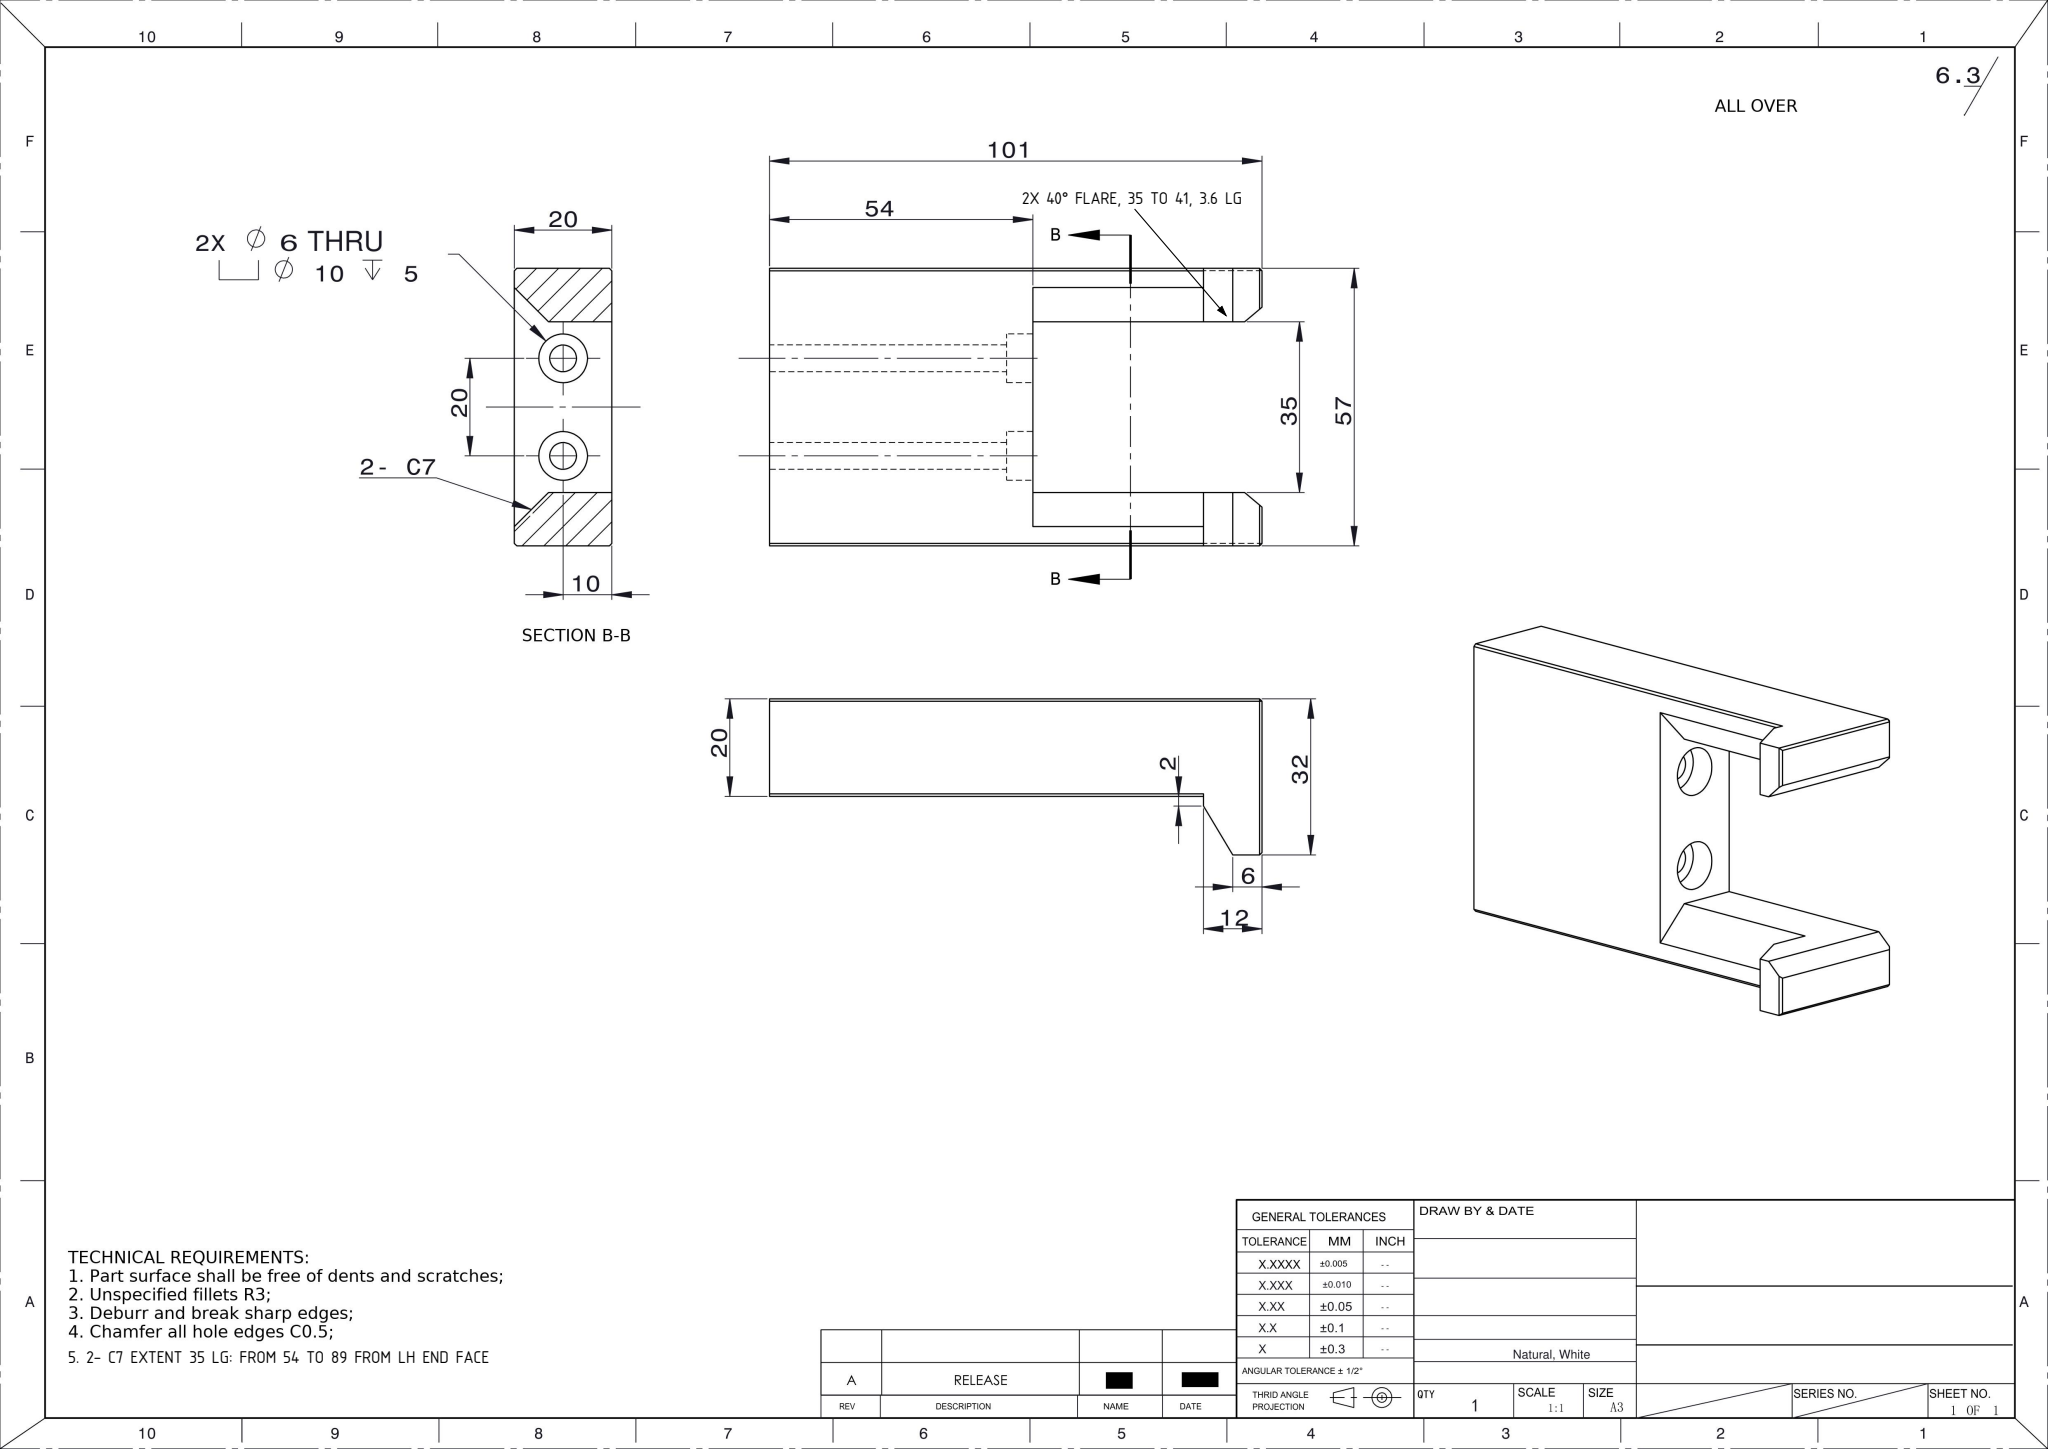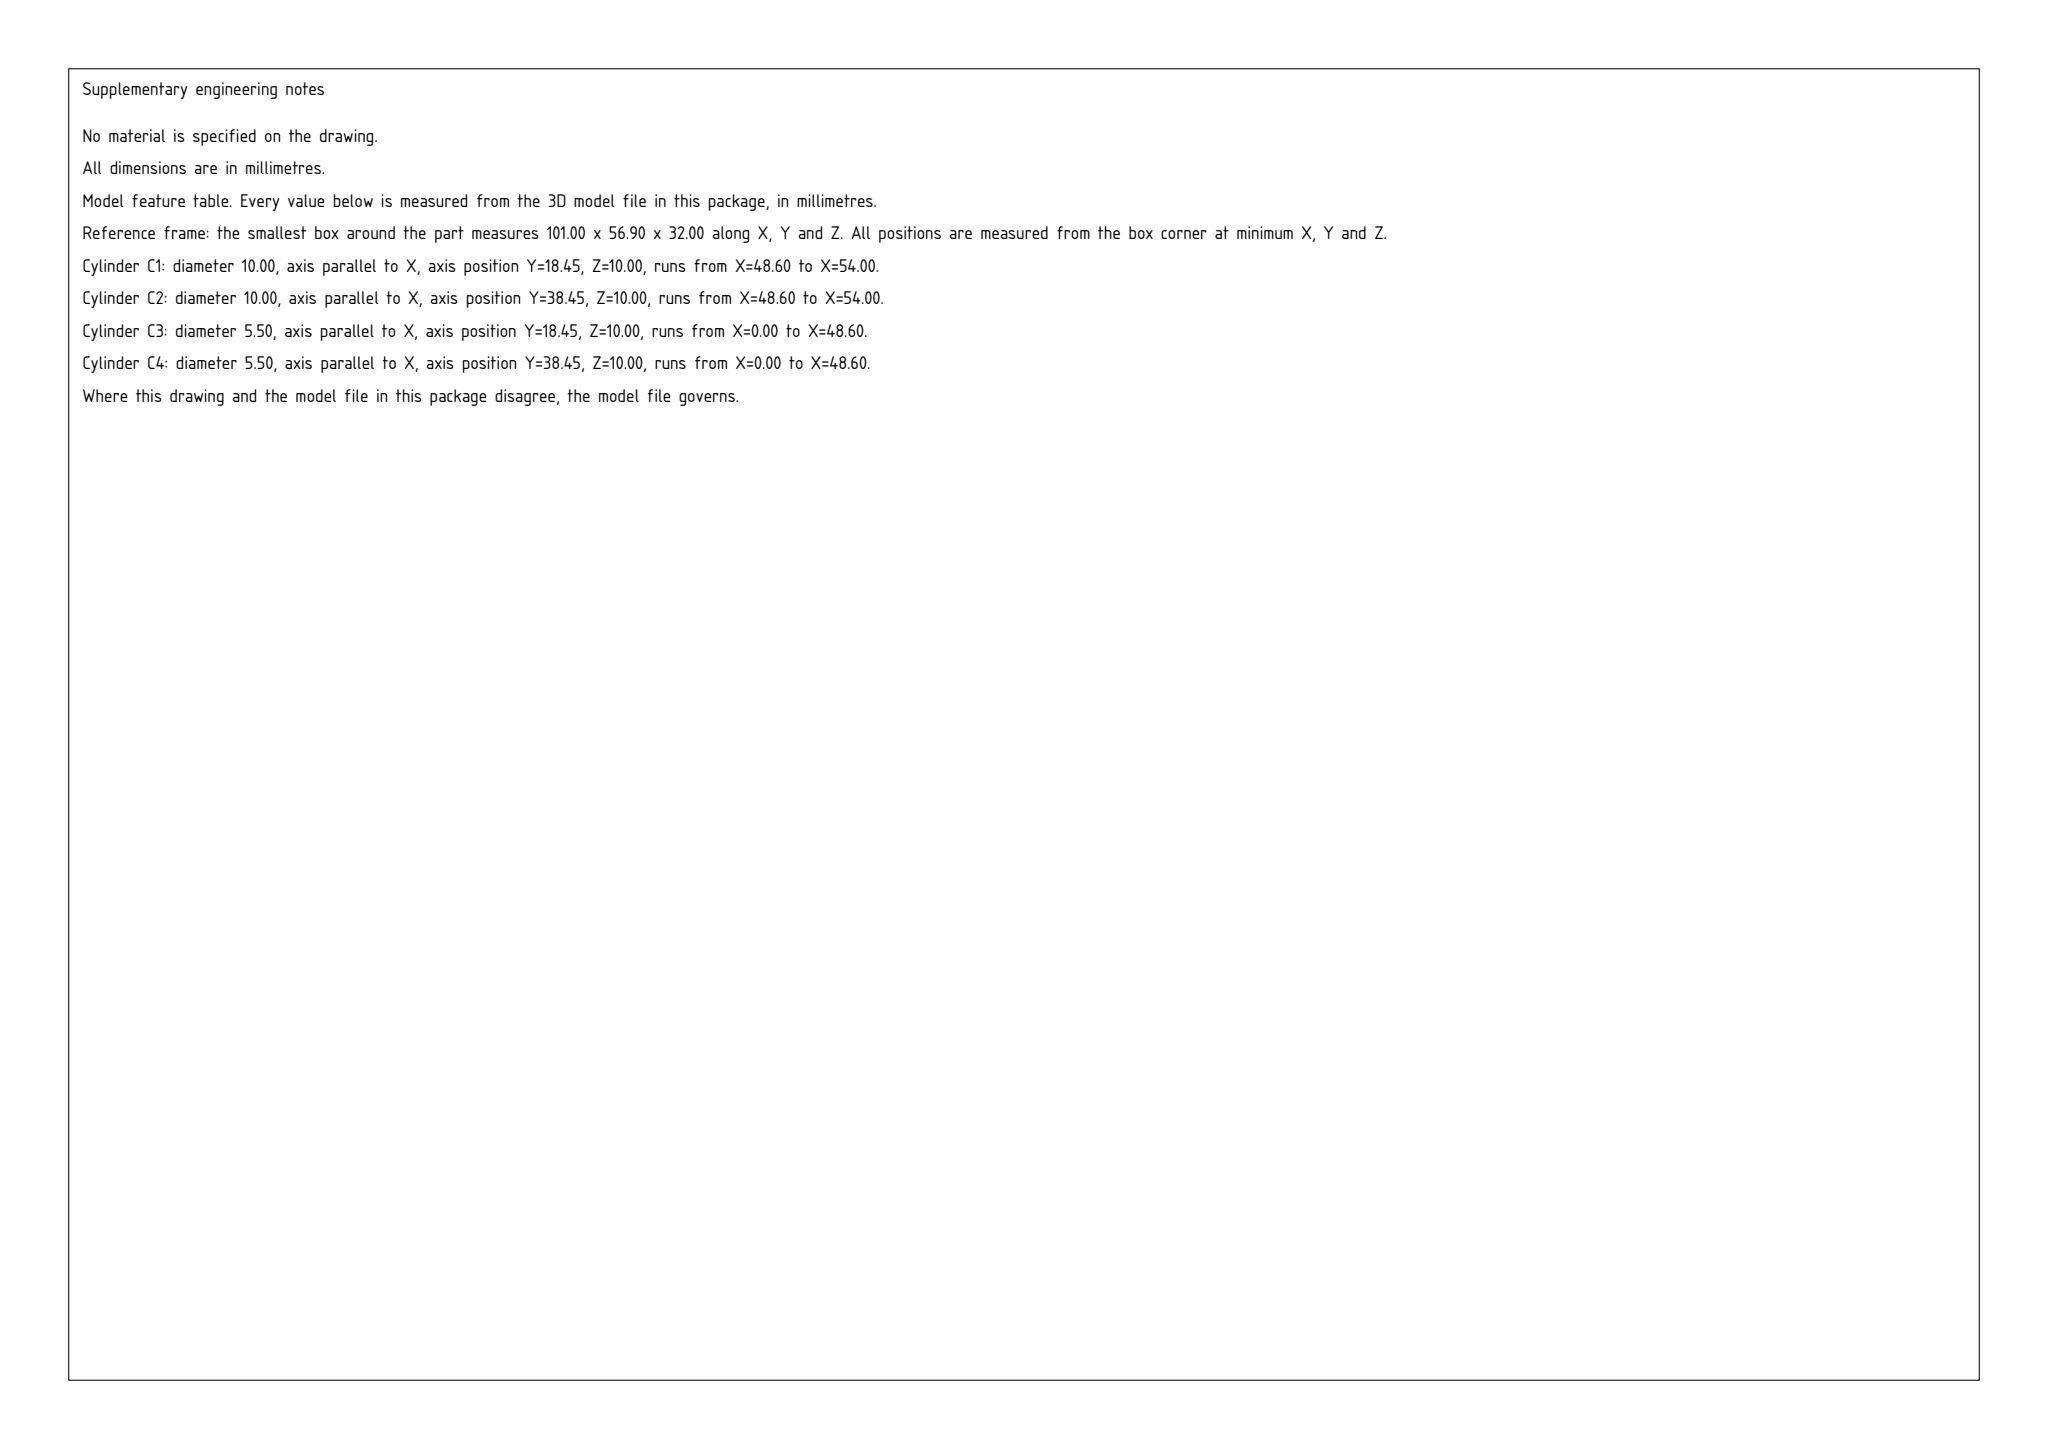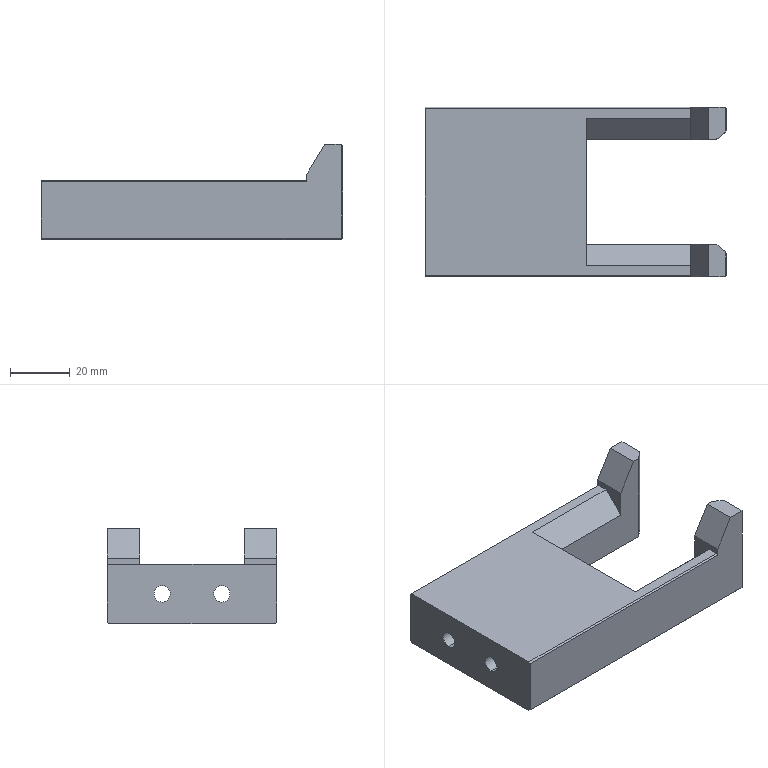Part | SolidWorks | mm | 1 solid | 42 faces | box 101 x 56.9 x 32 mm | volume 79260 mm3 | plane 34 | cylinder 8 | commonest cylinder face diameters 10 x4 5.5 x4
Drawing notes:
2X 40° FLARE OPENS 35 SLOT TO 41, 3.6 LG FROM RH END | from the solid: inclined planes 50/40/90 at bbox_from [97.4,8.0,0] and [97.4,46.0,0], size [3.6,3.0,32]; slot faces y=11/46 (35 wide) open to y=8/49 (41) at x=101 end
2- C7 EXTENT 35 LG: FROM 54 TO 89 FROM LH END FACE | from the solid: 45° chamfer planes bbox_from [54,4,13] and [54,46,13], size [35,7,7]; starts at slot bottom face x=54, ends at arm step x=89 (z=20 face ends x=89)
build123d program:
from build123d import *
from OCP.BRepFilletAPI import BRepFilletAPI_MakeChamfer

# Parameters (mm, degrees)
SKETCH1_W                                       = 89
SKETCH1_H                                       = 56.9
BOSS_EXTRUDE1_DEPTH                             = 20
SKETCH2_W                                       = 20
SKETCH2_H                                       = 35
CUT_EXTRUDE1_DEPTH                              = 35
CHAMFER1_SIZE                                   = 7
SKETCH3_W                                       = 32
SKETCH3_H                                       = 10.95
BOSS_EXTRUDE2_DEPTH                             = 12
CUT_EXTRUDE2_DEPTH                              = 95.121
M5_HEX_SOCKET_HEAD_CAP_SCREW_CBORE2_D           = 5.5
M5_HEX_SOCKET_HEAD_CAP_SCREW_CBORE2_CBORE_D     = 10
M5_HEX_SOCKET_HEAD_CAP_SCREW_CBORE2_CBORE_DEPTH = 5.4
CHAMFER2_SIZE                                   = 3
CHAMFER2_SIZE2                                  = 3.575
CHAMFER3_SIZE                                   = 0.5


with BuildPart() as part:
    # Sketch1 → Boss-Extrude1 (new body)
    with BuildSketch(Plane.XY):
        with Locations((11.302, -12.436)):
            Rectangle(SKETCH1_W, SKETCH1_H)
    extrude(amount=BOSS_EXTRUDE1_DEPTH)

    # Sketch2 → Cut-Extrude1 (cut)
    with BuildSketch(Plane(origin=(55.802, 0, 0), x_dir=(0, 0, -1), z_dir=(1, 0, 0))):
        with Locations((-10, -12.436)):
            Rectangle(SKETCH2_W, SKETCH2_H)
    extrude(amount=-CUT_EXTRUDE1_DEPTH, mode=Mode.SUBTRACT)

    # Chamfer1
    chamfer1_edges = [part.edges().sort_by_distance(p)[0] for p in [
        (38.302, -29.936, 20),
        (38.302, 5.064, 20),
    ]]
    chamfer(chamfer1_edges, length=CHAMFER1_SIZE)

    # Sketch3 → Boss-Extrude2 (add)
    with BuildSketch(Plane(origin=(55.802, 0, 0), x_dir=(0, 0, -1), z_dir=(1, 0, 0))):
        with Locations((-16, -35.411)):
            Rectangle(SKETCH3_W, SKETCH3_H)
        with Locations((-16, 10.539)):
            Rectangle(SKETCH3_W, SKETCH3_H)
    extrude(amount=BOSS_EXTRUDE2_DEPTH)

    # Sketch4 → Cut-Extrude2 (cut, through all)
    with BuildSketch(Plane.XZ.offset(40.886)):
        Polygon((55.802, 32), (55.802, 22), (61.802, 32), align=None)
    extrude(amount=-CUT_EXTRUDE2_DEPTH, mode=Mode.SUBTRACT)

    # M5 Hex Socket Head Cap Screw CBORE2 (through all)
    with Locations(Plane(origin=(20.802, 0, 0), x_dir=(0, 0, -1), z_dir=(1, 0, 0))):
        with Locations((-10, -2.436), (-10, -22.436)):
            CounterBoreHole(M5_HEX_SOCKET_HEAD_CAP_SCREW_CBORE2_D / 2, M5_HEX_SOCKET_HEAD_CAP_SCREW_CBORE2_CBORE_D / 2, M5_HEX_SOCKET_HEAD_CAP_SCREW_CBORE2_CBORE_DEPTH)

    # Chamfer2: one chamfer whose edges measure the first distance from different faces: ONE call of the kernel's chamfer builder (chamfer() names one face for all edges)
    chamfer2_edges_1 = [part.edges().sort_by_distance(p)[0] for p in [
        (67.802, -29.936, 16),
    ]]
    chamfer2_side_1 = [part.faces().sort_by_distance(p)[0] for p in [
        (67.802, -35.411, 16),
    ]]
    chamfer2_edges_2 = [part.edges().sort_by_distance(p)[0] for p in [
        (67.802, 5.064, 16),
    ]]
    chamfer2_side_2 = [part.faces().sort_by_distance(p)[0] for p in [
        (67.802, 10.539, 16),
    ]]
    chamfer2 = BRepFilletAPI_MakeChamfer(part.part.solid().wrapped)
    for e in chamfer2_edges_1:
        chamfer2.Add(CHAMFER2_SIZE, CHAMFER2_SIZE2, e.wrapped, chamfer2_side_1[0].wrapped)  # the first distance lies on this face
    for e in chamfer2_edges_2:
        chamfer2.Add(CHAMFER2_SIZE, CHAMFER2_SIZE2, e.wrapped, chamfer2_side_2[0].wrapped)  # the first distance lies on this face
    add(Compound.cast(chamfer2.Shape()), mode=Mode.REPLACE)

    # Chamfer3
    chamfer3_edges = [part.edges().sort_by_distance(p)[0] for p in [
        (67.802, -36.911, 32),
        (67.802, 12.039, 0),
        (11.302, 16.014, 20),
        (17.302, 16.014, 0),
        (67.802, -36.911, 0),
        (67.802, -40.886, 16),
        (17.302, -40.886, 0),
        (67.802, 16.014, 16),
        (67.802, 12.039, 32),
        (11.302, -40.886, 20),
    ]]
    chamfer(chamfer3_edges, length=CHAMFER3_SIZE)


solid = part.part